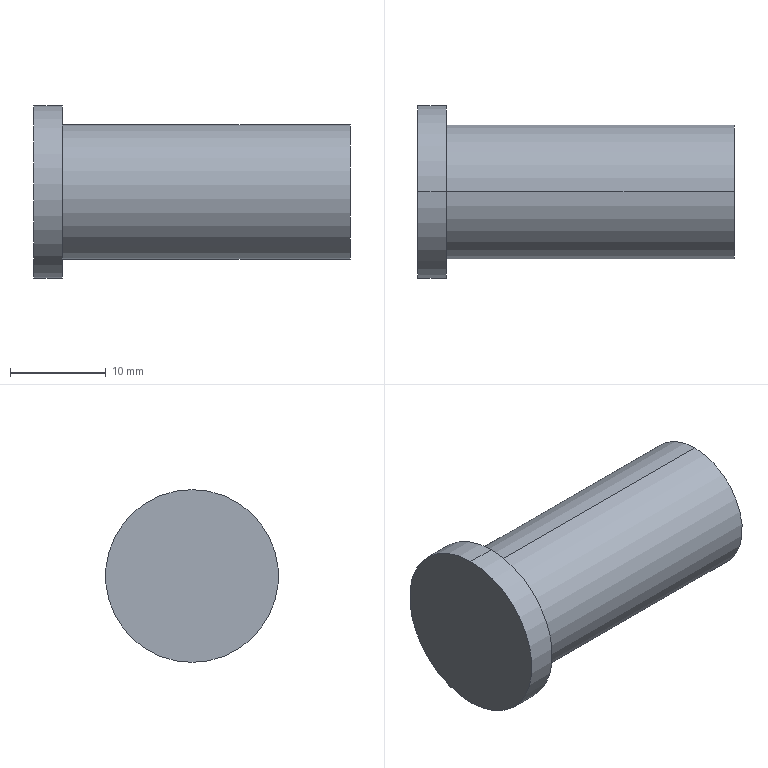Component | SolidWorks | 7mmScrew-10 | 1 solid | 7 faces | box 33 x 18 x 18 mm | volume 5382 mm3 | cylinder 4 | plane 3 | commonest cylinder face diameters 14 x2 18 x2
build123d program:
from build123d import *

# Parameters (mm, degrees)
SKETCH1_R           = 9
BOSS_EXTRUDE1_DEPTH = 3
SKETCH2_R           = 7
BOSS_EXTRUDE2_DEPTH = 30


with BuildPart() as part:
    # Sketch1 → Boss-Extrude1 (new body)
    with BuildSketch(Plane.XY):
        Circle(SKETCH1_R)
    extrude(amount=BOSS_EXTRUDE1_DEPTH)

    # Sketch2 → Boss-Extrude2 (add)
    with BuildSketch(Plane.XY.offset(3)):
        Circle(SKETCH2_R)
    extrude(amount=BOSS_EXTRUDE2_DEPTH)


solid = part.part

# Placed as in the assembly
solid = solid.moved(Location((102.641, -16.837, 0), (0, 90, 0)))